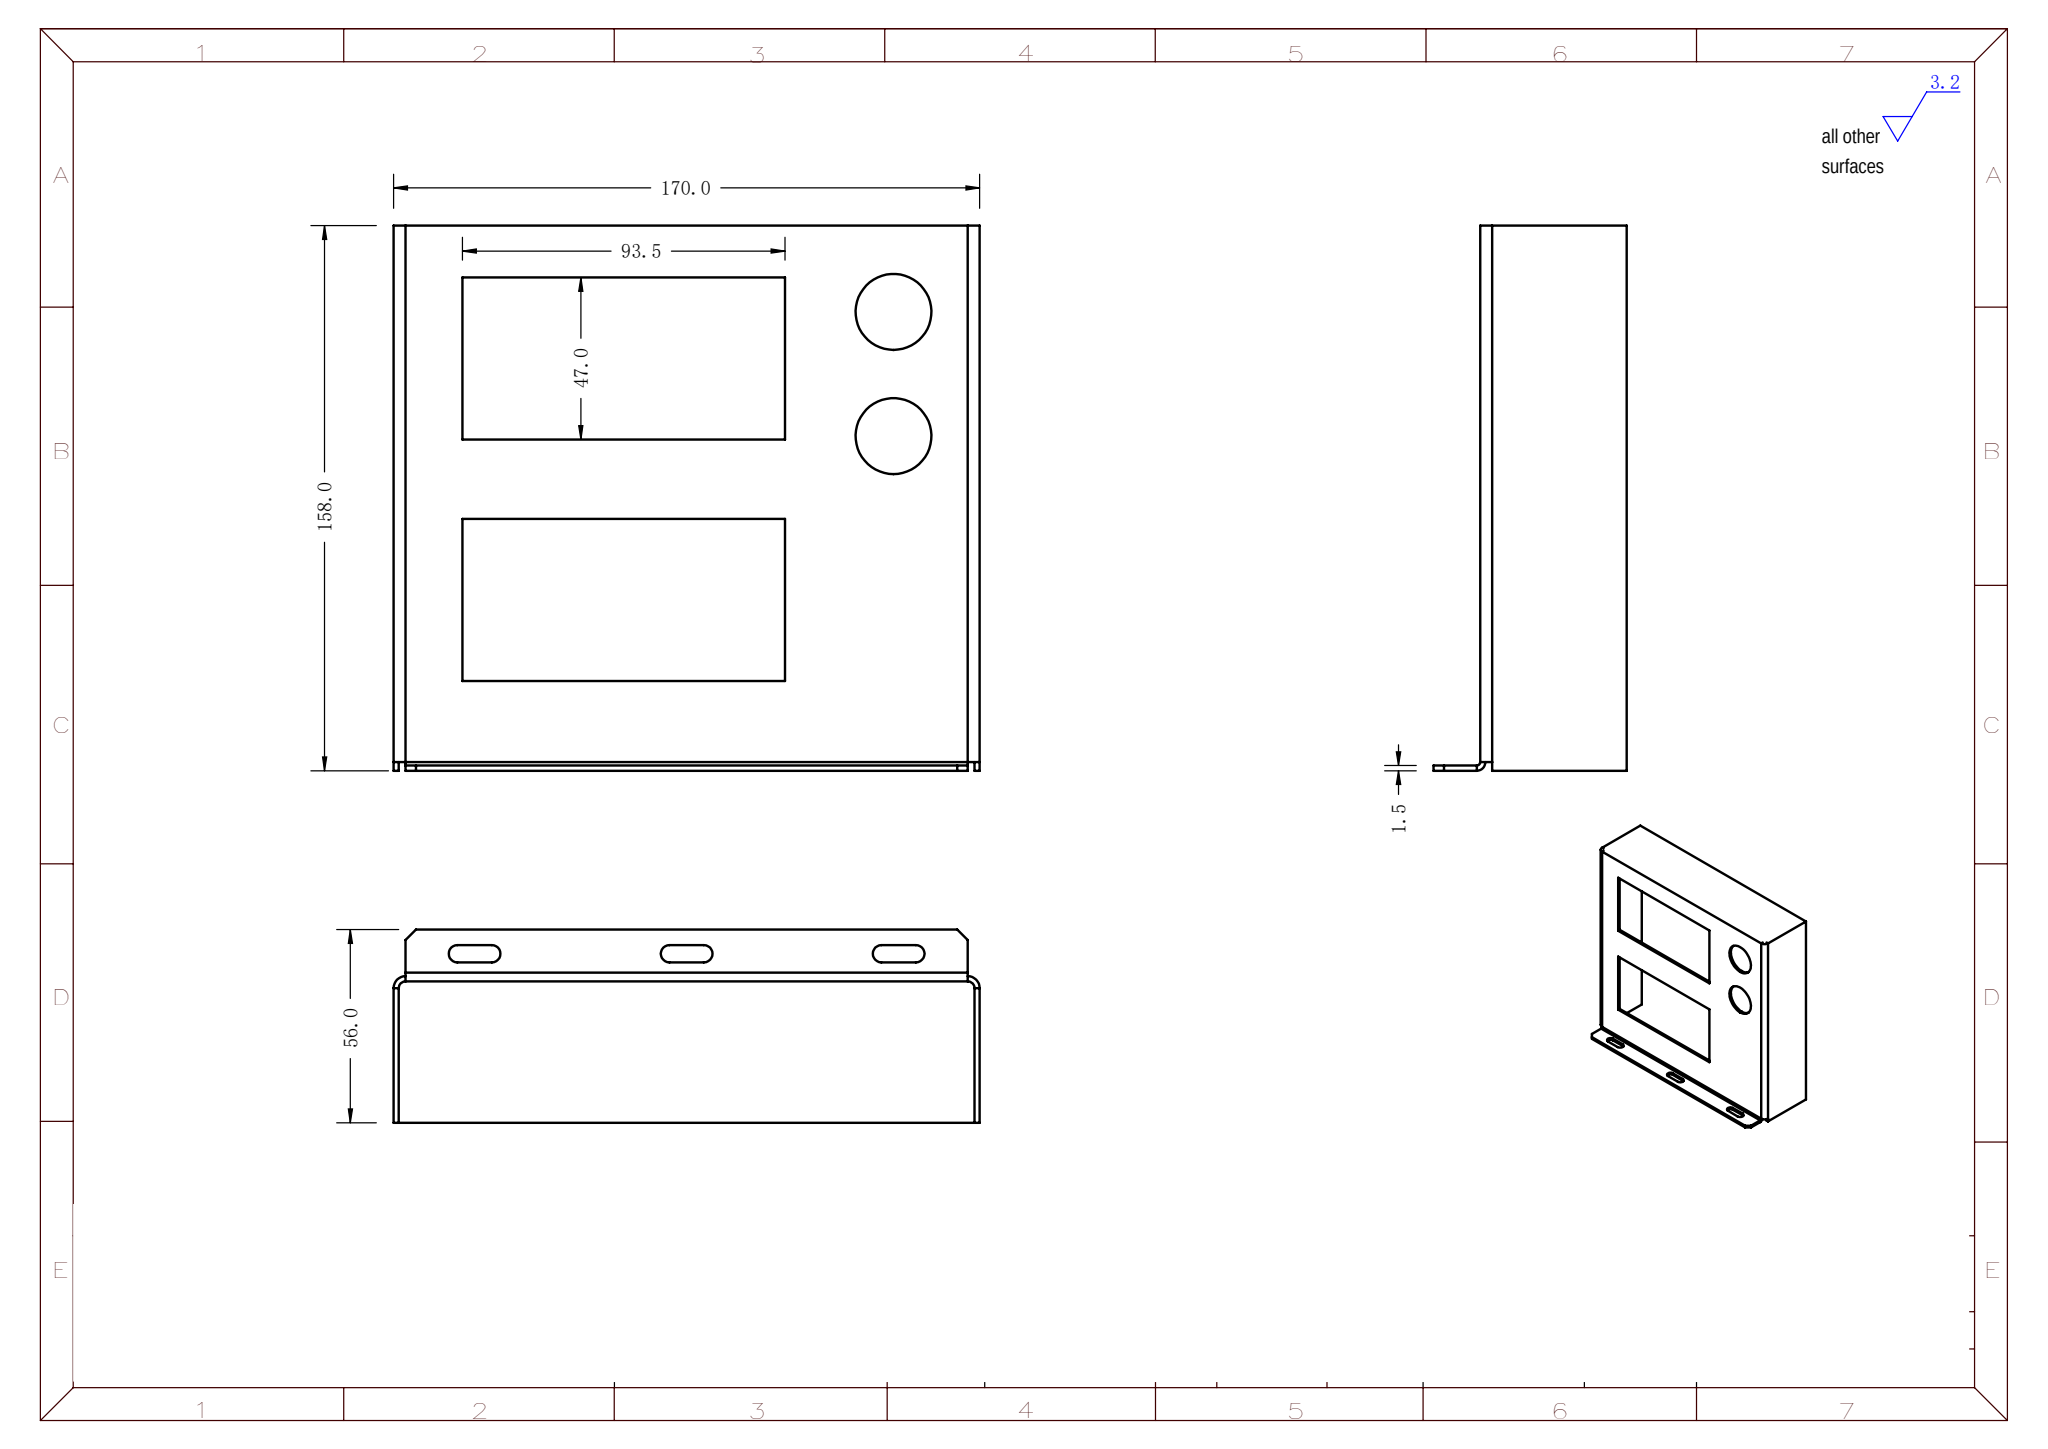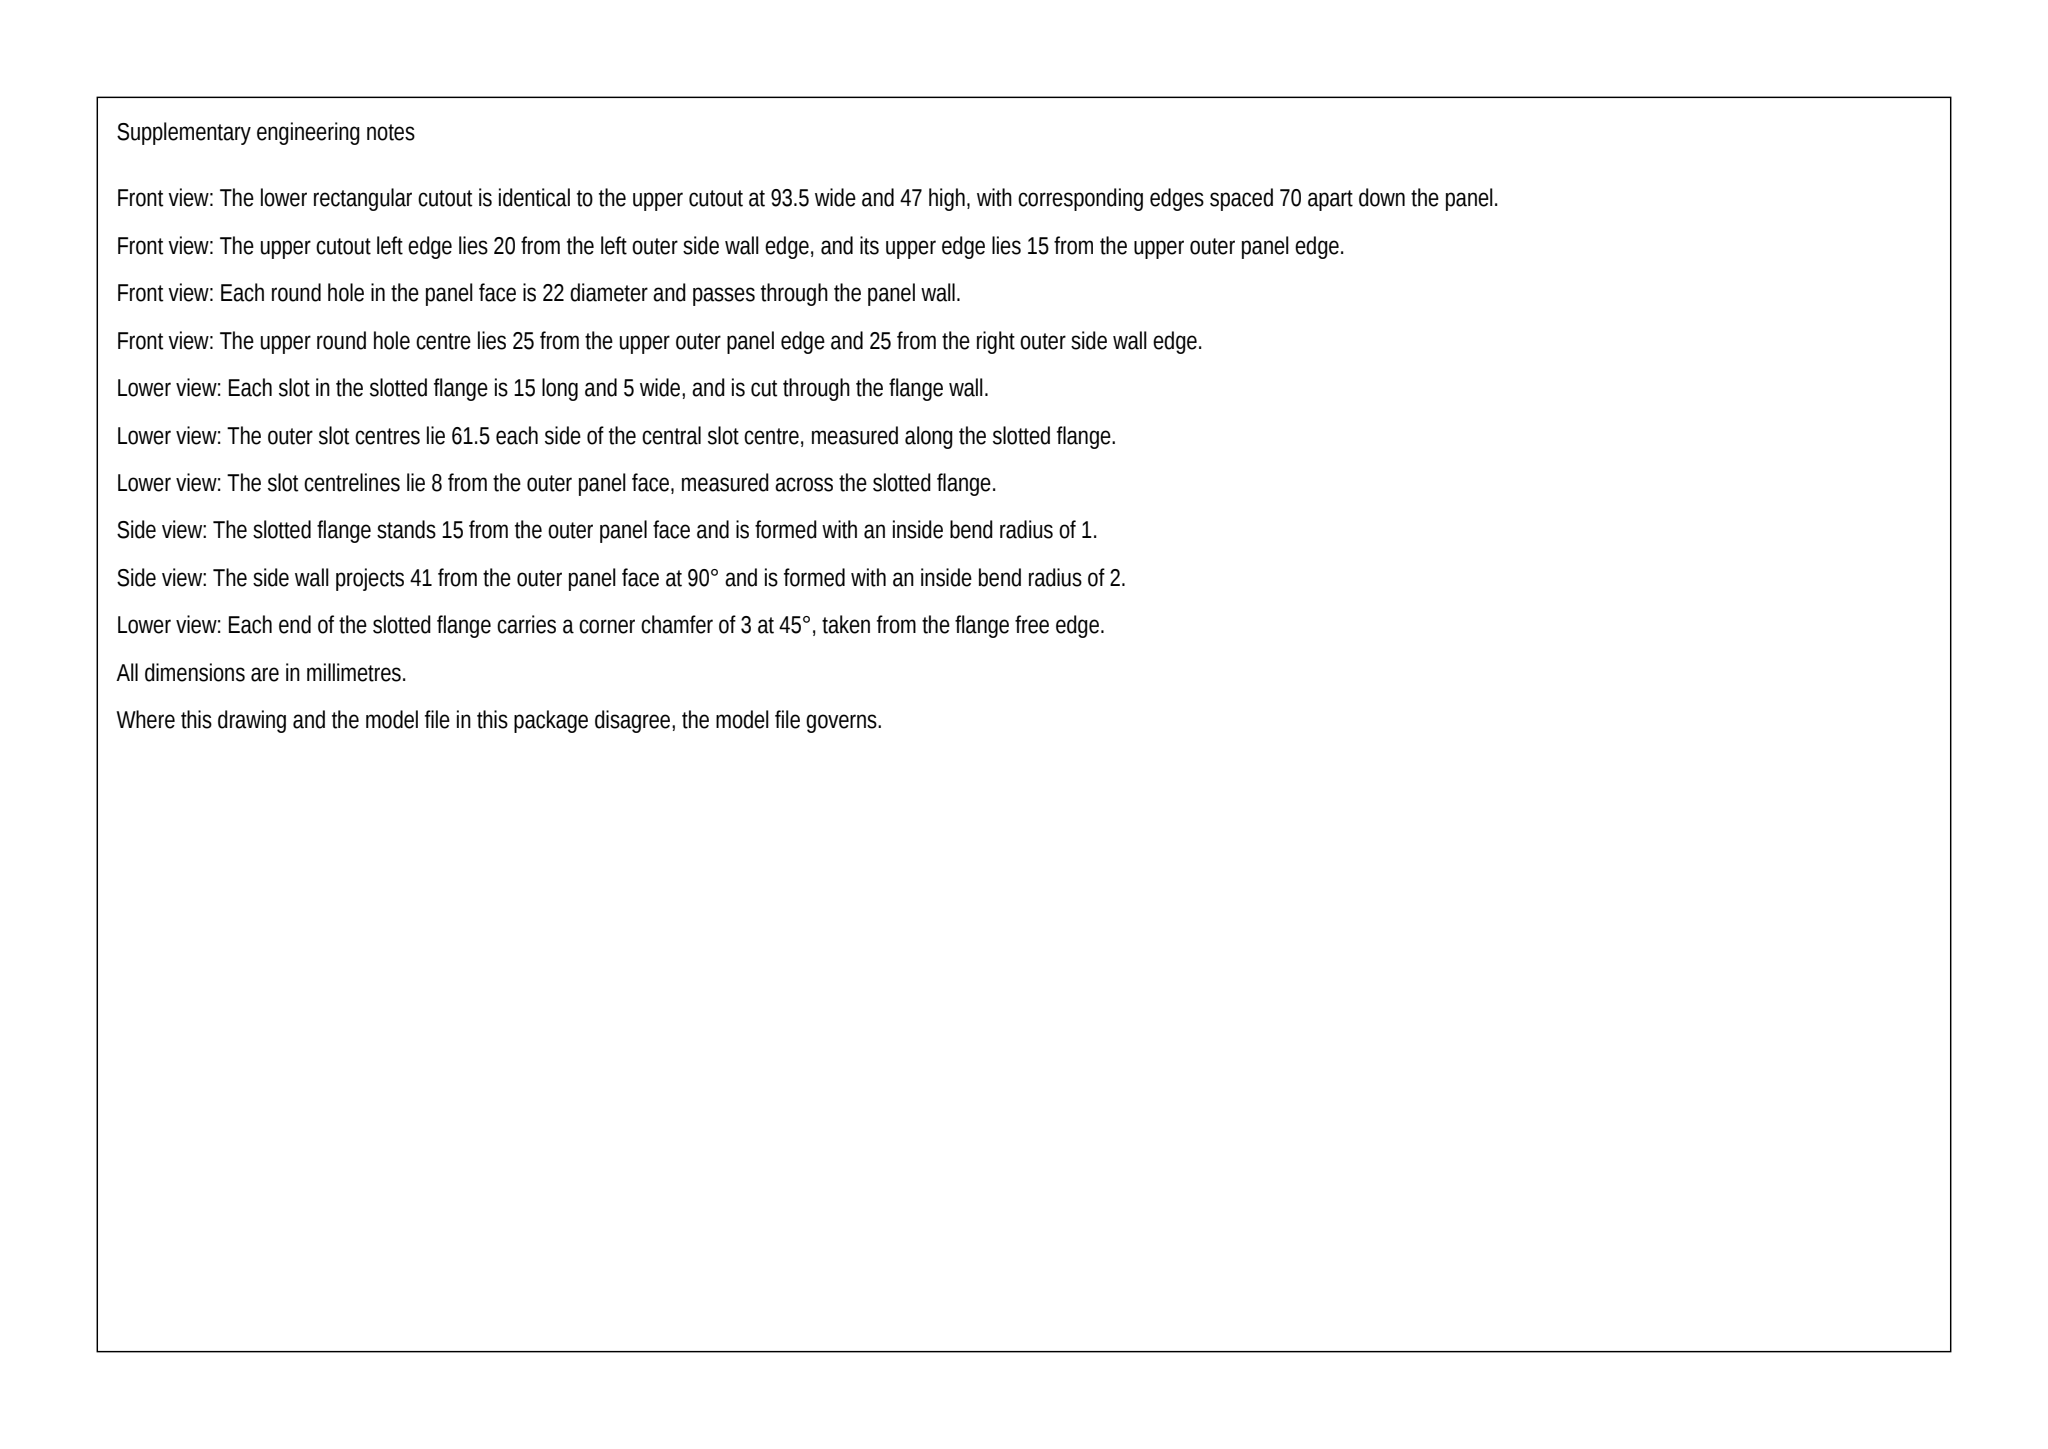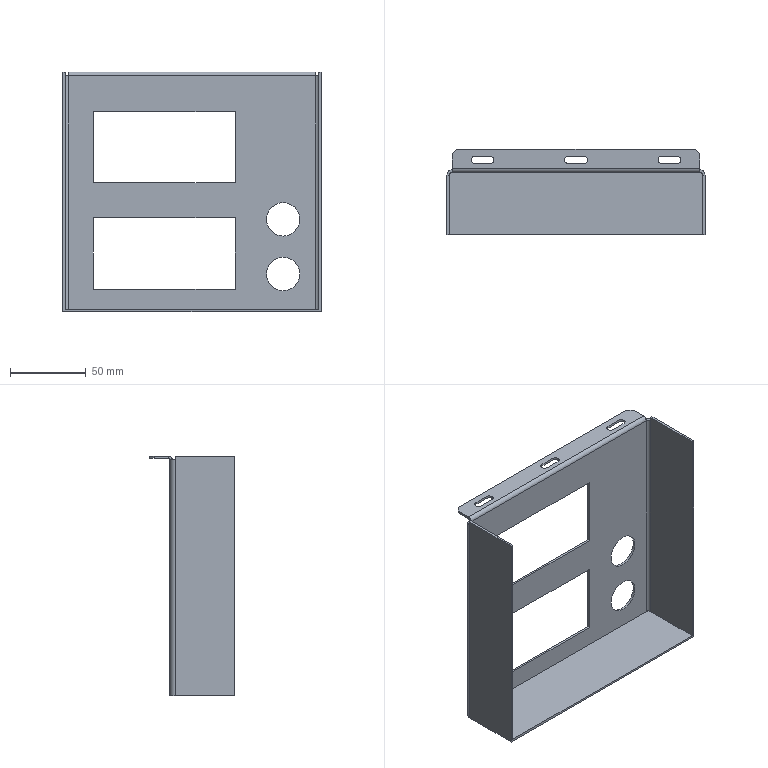Part | SolidWorks | mm | 1 solid | 57 faces | box 170 x 56 x 158 mm | volume 57866 mm3 | plane 38 | cylinder 19 | commonest cylinder face diameters 5 x10 22 x4 4 x2 7 x2 2 x1
Drawing notes:
OVERALL DEPTH 56.0 (FACE TO FLANGE REAR) | from the solid: bbox_xyz y = 56.0; y planes 0.0 thru 56.0
LOWER 93.5 X 47.0 POCKET 85.0 FROM TOP EDGE | from the solid: z planes 85.0 & 132.0, top edge datum z=0